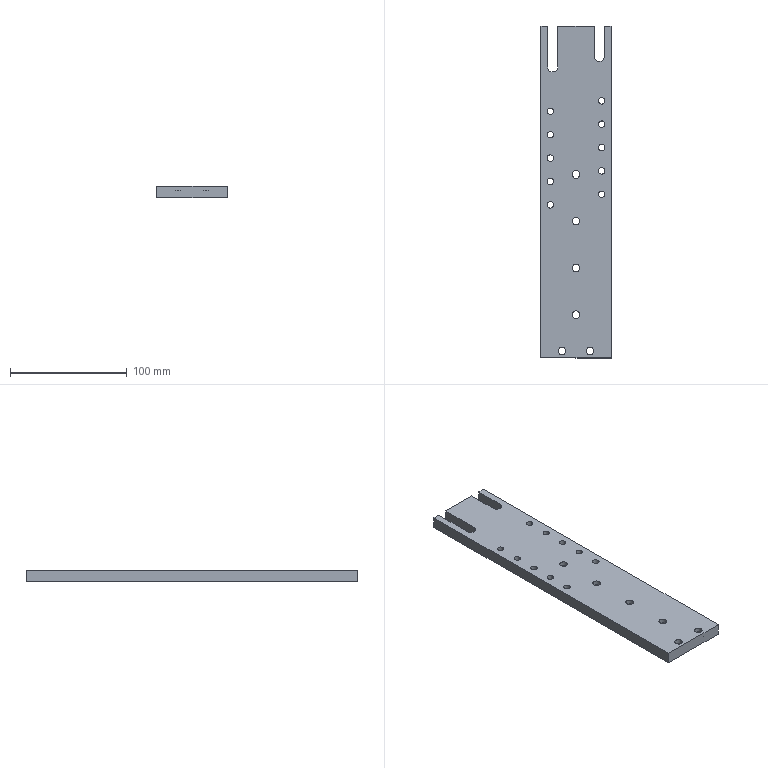Component | SolidWorks | 6GuidePlateH9.26-3 | 1 solid | 64 faces | box 60 x 284 x 10 mm | volume 158029 mm3 | cylinder 46 | plane 18 | commonest cylinder face diameters 5.5 x20 6.5 x12 11 x12 8.5 x2
build123d program:
from build123d import *

# Parameters (mm, degrees)
SKETCH1_W           = 60
SKETCH1_H           = 284
BOSS_EXTRUDE1_DEPTH = 10
SKETCH2_R           = 5.5
CUT_EXTRUDE1_DEPTH  = 6.2
SKETCH3_R           = 3.25
CUT_EXTRUDE2_DEPTH  = 291.335
SKETCH4_R           = 5.5
CUT_EXTRUDE3_DEPTH  = 6
SKETCH5_R           = 3.25
CUT_EXTRUDE4_DEPTH  = 291.331
SKETCH7_R           = 2.75
CUT_EXTRUDE6_DEPTH  = 291.441
CUT_EXTRUDE7_DEPTH  = 291.441


with BuildPart() as part:
    # Sketch1 → Boss-Extrude1 (new body)
    with BuildSketch(Plane.XY):
        with Locations((30, -142)):
            Rectangle(SKETCH1_W, SKETCH1_H)
    extrude(amount=BOSS_EXTRUDE1_DEPTH)

    # Sketch2 → Cut-Extrude1 (cut)
    with BuildSketch(Plane.XY.offset(10)):
        with Locations((18, -278)):
            Circle(SKETCH2_R)
        with Locations((42, -278)):
            Circle(SKETCH2_R)
    extrude(amount=-CUT_EXTRUDE1_DEPTH, mode=Mode.SUBTRACT)

    # Sketch3 → Cut-Extrude2 (cut, through all)
    with BuildSketch(Plane.XY.offset(3.8)):
        with Locations((18, -278)):
            Circle(SKETCH3_R)
        with Locations((42, -278)):
            Circle(SKETCH3_R)
    extrude(amount=-CUT_EXTRUDE2_DEPTH, mode=Mode.SUBTRACT)

    # Sketch4 → Cut-Extrude3 (cut)
    with BuildSketch(Plane.XY.offset(10)):
        with Locations((30, -247)):
            Circle(SKETCH4_R)
        with Locations((30, -207)):
            Circle(SKETCH4_R)
        with Locations((30, -167)):
            Circle(SKETCH4_R)
        with Locations((30, -127)):
            Circle(SKETCH4_R)
    extrude(amount=-CUT_EXTRUDE3_DEPTH, mode=Mode.SUBTRACT)

    # Sketch5 → Cut-Extrude4 (cut, through all)
    with BuildSketch(Plane.XY.offset(4)):
        with Locations((30, -247)):
            Circle(SKETCH5_R)
        with Locations((30, -207)):
            Circle(SKETCH5_R)
        with Locations((30, -167)):
            Circle(SKETCH5_R)
        with Locations((30, -127)):
            Circle(SKETCH5_R)
    extrude(amount=-CUT_EXTRUDE4_DEPTH, mode=Mode.SUBTRACT)

    # Sketch7 → Cut-Extrude6 (cut, through all)
    with BuildSketch(Plane(origin=(0, 0, 0), x_dir=(-1, 0, 0), z_dir=(0, 0, -1))):
        with Locations((-52, -153)):
            Circle(SKETCH7_R)
        with Locations((-8, -144)):
            Circle(SKETCH7_R)
        with Locations((-52, -133)):
            Circle(SKETCH7_R)
        with Locations((-8, -124)):
            Circle(SKETCH7_R)
        with Locations((-52, -113)):
            Circle(SKETCH7_R)
        with Locations((-8, -104)):
            Circle(SKETCH7_R)
        with Locations((-52, -93)):
            Circle(SKETCH7_R)
        with Locations((-8, -84)):
            Circle(SKETCH7_R)
        with Locations((-52, -73)):
            Circle(SKETCH7_R)
        with Locations((-8, -64)):
            Circle(SKETCH7_R)
    extrude(amount=-CUT_EXTRUDE6_DEPTH, mode=Mode.SUBTRACT)

    # Sketch8 → Cut-Extrude7 (cut, through all)
    with BuildSketch(Plane(origin=(0, 0, 0), x_dir=(-1, 0, 0), z_dir=(0, 0, -1))):
        with BuildLine():
            Line((-54.25, -35), (-54.25, 6.839))
            ThreePointArc((-54.25, 6.839), (-50, 11.089), (-45.75, 6.839))
            Line((-45.75, 6.839), (-45.75, -35))
            ThreePointArc((-45.75, -35), (-50, -39.25), (-54.25, -35))
        make_face()
        with BuildLine():
            Line((-14.25, -26), (-14.25, 4.932))
            ThreePointArc((-14.25, 4.932), (-10, 9.182), (-5.75, 4.932))
            Line((-5.75, 4.932), (-5.75, -26))
            ThreePointArc((-5.75, -26), (-10, -30.25), (-14.25, -26))
        make_face()
    extrude(amount=-CUT_EXTRUDE7_DEPTH, mode=Mode.SUBTRACT)


solid = part.part

# Placed as in the assembly
solid = solid.moved(Location((286, 109, 40.5), (-180, 0, 180)))